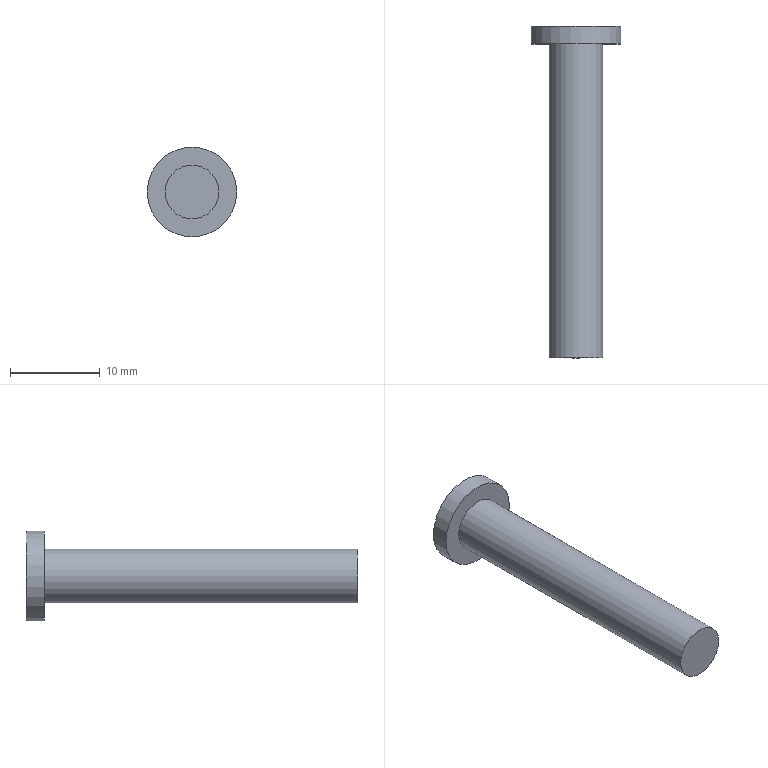Component | NX | SHE_JI-5 | 1 solid | 5 faces | box 10 x 37 x 10 mm | volume 1147 mm3 | plane 3 | cylinder 2 | commonest cylinder face diameters 6 x1 10 x1
STEP:
#1=CARTESIAN_POINT('',(0.,0.,0.));
#2=DIRECTION('',(0.,0.,1.));
#3=DIRECTION('',(1.,0.,0.));
#4=AXIS2_PLACEMENT_3D('',#1,#2,#3);
#5=CARTESIAN_POINT('',(-45.,-19.,20.));
#6=VERTEX_POINT('',#5);
#7=CARTESIAN_POINT('',(-48.,-19.,20.));
#8=DIRECTION('',(0.,1.,0.));
#9=DIRECTION('',(1.,0.,0.));
#10=AXIS2_PLACEMENT_3D('',#7,#8,#9);
#11=CIRCLE('',#10,3.);
#12=CARTESIAN_POINT('',(-48.,-19.,20.));
#13=DIRECTION('',(0.,-1.,0.));
#14=DIRECTION('',(1.,0.,0.));
#15=AXIS2_PLACEMENT_3D('',#12,#13,#14);
#16=PLANE('',#15);
#17=CARTESIAN_POINT('',(3.,0.));
#18=CARTESIAN_POINT('',(3.,-5.196));
#19=CARTESIAN_POINT('',(-1.5,-2.598));
#20=CARTESIAN_POINT('',(-6.,-0.));
#21=CARTESIAN_POINT('',(-1.5,2.598));
#22=CARTESIAN_POINT('',(3.,5.196));
#23=CARTESIAN_POINT('',(3.,0.));
#24=(BOUNDED_CURVE()B_SPLINE_CURVE(2,(#17,#18,#19,#20,#21,#22,#23),.UNSPECIFIED.,.T.,.F.)B_SPLINE_CURVE_WITH_KNOTS((1,2,2,2,2,1),(-2.094,0.,2.094,4.189,6.283,8.378),.UNSPECIFIED.)CURVE()GEOMETRIC_REPRESENTATION_ITEM()RATIONAL_B_SPLINE_CURVE((1.,0.5,1.,0.5,1.,0.5,1.))REPRESENTATION_ITEM(''));
#25=(GEOMETRIC_REPRESENTATION_CONTEXT(2)PARAMETRIC_REPRESENTATION_CONTEXT()REPRESENTATION_CONTEXT('',''));
#26=DEFINITIONAL_REPRESENTATION('',(#24),#25);
#27=PCURVE('',#16,#26);
#28=CARTESIAN_POINT('',(-48.,16.,20.));
#29=DIRECTION('',(0.,-1.,0.));
#30=DIRECTION('',(1.,0.,0.));
#31=AXIS2_PLACEMENT_3D('',#28,#29,#30);
#32=CYLINDRICAL_SURFACE('',#31,3.);
#33=CARTESIAN_POINT('',(6.283,35.));
#34=DIRECTION('',(-1.,0.));
#35=VECTOR('',#34,1.);
#36=LINE('',#33,#35);
#37=(GEOMETRIC_REPRESENTATION_CONTEXT(2)PARAMETRIC_REPRESENTATION_CONTEXT()REPRESENTATION_CONTEXT('',''));
#38=DEFINITIONAL_REPRESENTATION('',(#36),#37);
#39=PCURVE('',#32,#38);
#40=SURFACE_CURVE('',#11,(#27,#39),.PCURVE_S1.);
#41=EDGE_CURVE('',#6,#6,#40,.T.);
#42=ORIENTED_EDGE('',*,*,#41,.F.);
#43=EDGE_LOOP('',(#42));
#44=FACE_BOUND('',#43,.T.);
#45=ADVANCED_FACE('',(#44),#16,.T.);
#46=ORIENTED_EDGE('',*,*,#41,.T.);
#47=CARTESIAN_POINT('',(-45.,16.,20.));
#48=VERTEX_POINT('',#47);
#49=CARTESIAN_POINT('',(-45.,16.,20.));
#50=CARTESIAN_POINT('',(-45.,-19.,20.));
#51=B_SPLINE_CURVE_WITH_KNOTS('',1,(#49,#50),.UNSPECIFIED.,.F.,.F.,(2,2),(0.,35.),.PIECEWISE_BEZIER_KNOTS.);
#52=CARTESIAN_POINT('',(0.,0.));
#53=DIRECTION('',(0.,1.));
#54=VECTOR('',#53,1.);
#55=LINE('',#52,#54);
#56=(GEOMETRIC_REPRESENTATION_CONTEXT(2)PARAMETRIC_REPRESENTATION_CONTEXT()REPRESENTATION_CONTEXT('',''));
#57=DEFINITIONAL_REPRESENTATION('',(#55),#56);
#58=PCURVE('',#32,#57);
#59=CARTESIAN_POINT('',(6.283,0.));
#60=DIRECTION('',(0.,1.));
#61=VECTOR('',#60,1.);
#62=LINE('',#59,#61);
#63=(GEOMETRIC_REPRESENTATION_CONTEXT(2)PARAMETRIC_REPRESENTATION_CONTEXT()REPRESENTATION_CONTEXT('',''));
#64=DEFINITIONAL_REPRESENTATION('',(#62),#63);
#65=PCURVE('',#32,#64);
#66=SEAM_CURVE('',#51,(#58,#65),.PCURVE_S1.);
#67=EDGE_CURVE('',#48,#6,#66,.T.);
#68=ORIENTED_EDGE('',*,*,#67,.F.);
#69=CARTESIAN_POINT('',(-48.,16.,20.));
#70=DIRECTION('',(0.,-1.,0.));
#71=DIRECTION('',(1.,0.,0.));
#72=AXIS2_PLACEMENT_3D('',#69,#70,#71);
#73=CIRCLE('',#72,3.);
#74=CARTESIAN_POINT('',(0.,0.));
#75=DIRECTION('',(1.,0.));
#76=VECTOR('',#75,1.);
#77=LINE('',#74,#76);
#78=(GEOMETRIC_REPRESENTATION_CONTEXT(2)PARAMETRIC_REPRESENTATION_CONTEXT()REPRESENTATION_CONTEXT('',''));
#79=DEFINITIONAL_REPRESENTATION('',(#77),#78);
#80=PCURVE('',#32,#79);
#81=CARTESIAN_POINT('',(-48.,16.,20.));
#82=DIRECTION('',(0.,-1.,0.));
#83=DIRECTION('',(1.,0.,0.));
#84=AXIS2_PLACEMENT_3D('',#81,#82,#83);
#85=PLANE('',#84);
#86=CARTESIAN_POINT('',(0.,0.));
#87=DIRECTION('',(1.,0.));
#88=AXIS2_PLACEMENT_2D('',#86,#87);
#89=CIRCLE('',#88,3.);
#90=(GEOMETRIC_REPRESENTATION_CONTEXT(2)PARAMETRIC_REPRESENTATION_CONTEXT()REPRESENTATION_CONTEXT('',''));
#91=DEFINITIONAL_REPRESENTATION('',(#89),#90);
#92=PCURVE('',#85,#91);
#93=SURFACE_CURVE('',#73,(#80,#92),.PCURVE_S1.);
#94=EDGE_CURVE('',#48,#48,#93,.T.);
#95=ORIENTED_EDGE('',*,*,#94,.T.);
#96=ORIENTED_EDGE('',*,*,#67,.T.);
#97=EDGE_LOOP('',(#46,#68,#95,#96));
#98=FACE_BOUND('',#97,.T.);
#99=ADVANCED_FACE('',(#98),#32,.T.);
#100=CARTESIAN_POINT('',(-43.,18.,20.));
#101=VERTEX_POINT('',#100);
#102=CARTESIAN_POINT('',(-48.,18.,20.));
#103=DIRECTION('',(0.,-1.,0.));
#104=DIRECTION('',(1.,0.,0.));
#105=AXIS2_PLACEMENT_3D('',#102,#103,#104);
#106=CIRCLE('',#105,5.);
#107=CARTESIAN_POINT('',(-48.,18.,20.));
#108=DIRECTION('',(0.,1.,0.));
#109=DIRECTION('',(-1.,0.,0.));
#110=AXIS2_PLACEMENT_3D('',#107,#108,#109);
#111=PLANE('',#110);
#112=CARTESIAN_POINT('',(-5.,0.));
#113=CARTESIAN_POINT('',(-5.,8.66));
#114=CARTESIAN_POINT('',(2.5,4.33));
#115=CARTESIAN_POINT('',(10.,0.));
#116=CARTESIAN_POINT('',(2.5,-4.33));
#117=CARTESIAN_POINT('',(-5.,-8.66));
#118=CARTESIAN_POINT('',(-5.,0.));
#119=(BOUNDED_CURVE()B_SPLINE_CURVE(2,(#112,#113,#114,#115,#116,#117,#118),.UNSPECIFIED.,.T.,.F.)B_SPLINE_CURVE_WITH_KNOTS((1,2,2,2,2,1),(-2.094,0.,2.094,4.189,6.283,8.378),.UNSPECIFIED.)CURVE()GEOMETRIC_REPRESENTATION_ITEM()RATIONAL_B_SPLINE_CURVE((1.,0.5,1.,0.5,1.,0.5,1.))REPRESENTATION_ITEM(''));
#120=(GEOMETRIC_REPRESENTATION_CONTEXT(2)PARAMETRIC_REPRESENTATION_CONTEXT()REPRESENTATION_CONTEXT('',''));
#121=DEFINITIONAL_REPRESENTATION('',(#119),#120);
#122=PCURVE('',#111,#121);
#123=CARTESIAN_POINT('',(-48.,16.,20.));
#124=DIRECTION('',(0.,1.,0.));
#125=DIRECTION('',(1.,0.,0.));
#126=AXIS2_PLACEMENT_3D('',#123,#124,#125);
#127=CYLINDRICAL_SURFACE('',#126,5.);
#128=CARTESIAN_POINT('',(6.283,2.));
#129=DIRECTION('',(-1.,0.));
#130=VECTOR('',#129,1.);
#131=LINE('',#128,#130);
#132=(GEOMETRIC_REPRESENTATION_CONTEXT(2)PARAMETRIC_REPRESENTATION_CONTEXT()REPRESENTATION_CONTEXT('',''));
#133=DEFINITIONAL_REPRESENTATION('',(#131),#132);
#134=PCURVE('',#127,#133);
#135=SURFACE_CURVE('',#106,(#122,#134),.PCURVE_S1.);
#136=EDGE_CURVE('',#101,#101,#135,.T.);
#137=ORIENTED_EDGE('',*,*,#136,.F.);
#138=EDGE_LOOP('',(#137));
#139=FACE_BOUND('',#138,.T.);
#140=ADVANCED_FACE('',(#139),#111,.T.);
#141=ORIENTED_EDGE('',*,*,#94,.F.);
#142=EDGE_LOOP('',(#141));
#143=FACE_BOUND('',#142,.T.);
#144=CARTESIAN_POINT('',(-43.,16.,20.));
#145=VERTEX_POINT('',#144);
#146=CARTESIAN_POINT('',(-48.,16.,20.));
#147=DIRECTION('',(0.,1.,0.));
#148=DIRECTION('',(1.,0.,0.));
#149=AXIS2_PLACEMENT_3D('',#146,#147,#148);
#150=CIRCLE('',#149,5.);
#151=CARTESIAN_POINT('',(5.,0.));
#152=CARTESIAN_POINT('',(5.,-8.66));
#153=CARTESIAN_POINT('',(-2.5,-4.33));
#154=CARTESIAN_POINT('',(-10.,-0.));
#155=CARTESIAN_POINT('',(-2.5,4.33));
#156=CARTESIAN_POINT('',(5.,8.66));
#157=CARTESIAN_POINT('',(5.,0.));
#158=(BOUNDED_CURVE()B_SPLINE_CURVE(2,(#151,#152,#153,#154,#155,#156,#157),.UNSPECIFIED.,.T.,.F.)B_SPLINE_CURVE_WITH_KNOTS((1,2,2,2,2,1),(-2.094,0.,2.094,4.189,6.283,8.378),.UNSPECIFIED.)CURVE()GEOMETRIC_REPRESENTATION_ITEM()RATIONAL_B_SPLINE_CURVE((1.,0.5,1.,0.5,1.,0.5,1.))REPRESENTATION_ITEM(''));
#159=(GEOMETRIC_REPRESENTATION_CONTEXT(2)PARAMETRIC_REPRESENTATION_CONTEXT()REPRESENTATION_CONTEXT('',''));
#160=DEFINITIONAL_REPRESENTATION('',(#158),#159);
#161=PCURVE('',#85,#160);
#162=CARTESIAN_POINT('',(0.,0.));
#163=DIRECTION('',(1.,0.));
#164=VECTOR('',#163,1.);
#165=LINE('',#162,#164);
#166=(GEOMETRIC_REPRESENTATION_CONTEXT(2)PARAMETRIC_REPRESENTATION_CONTEXT()REPRESENTATION_CONTEXT('',''));
#167=DEFINITIONAL_REPRESENTATION('',(#165),#166);
#168=PCURVE('',#127,#167);
#169=SURFACE_CURVE('',#150,(#161,#168),.PCURVE_S1.);
#170=EDGE_CURVE('',#145,#145,#169,.T.);
#171=ORIENTED_EDGE('',*,*,#170,.F.);
#172=EDGE_LOOP('',(#171));
#173=FACE_BOUND('',#172,.T.);
#174=ADVANCED_FACE('',(#143,#173),#85,.T.);
#175=ORIENTED_EDGE('',*,*,#136,.T.);
#176=CARTESIAN_POINT('',(-43.,16.,20.));
#177=CARTESIAN_POINT('',(-43.,18.,20.));
#178=B_SPLINE_CURVE_WITH_KNOTS('',1,(#176,#177),.UNSPECIFIED.,.F.,.F.,(2,2),(0.,2.),.PIECEWISE_BEZIER_KNOTS.);
#179=CARTESIAN_POINT('',(0.,0.));
#180=DIRECTION('',(0.,1.));
#181=VECTOR('',#180,1.);
#182=LINE('',#179,#181);
#183=(GEOMETRIC_REPRESENTATION_CONTEXT(2)PARAMETRIC_REPRESENTATION_CONTEXT()REPRESENTATION_CONTEXT('',''));
#184=DEFINITIONAL_REPRESENTATION('',(#182),#183);
#185=PCURVE('',#127,#184);
#186=CARTESIAN_POINT('',(6.283,0.));
#187=DIRECTION('',(0.,1.));
#188=VECTOR('',#187,1.);
#189=LINE('',#186,#188);
#190=(GEOMETRIC_REPRESENTATION_CONTEXT(2)PARAMETRIC_REPRESENTATION_CONTEXT()REPRESENTATION_CONTEXT('',''));
#191=DEFINITIONAL_REPRESENTATION('',(#189),#190);
#192=PCURVE('',#127,#191);
#193=SEAM_CURVE('',#178,(#185,#192),.PCURVE_S1.);
#194=EDGE_CURVE('',#145,#101,#193,.T.);
#195=ORIENTED_EDGE('',*,*,#194,.F.);
#196=ORIENTED_EDGE('',*,*,#170,.T.);
#197=ORIENTED_EDGE('',*,*,#194,.T.);
#198=EDGE_LOOP('',(#175,#195,#196,#197));
#199=FACE_BOUND('',#198,.T.);
#200=ADVANCED_FACE('',(#199),#127,.T.);
#201=CLOSED_SHELL('',(#45,#99,#140,#174,#200));
#202=MANIFOLD_SOLID_BREP('',#201);
#203=(LENGTH_UNIT()NAMED_UNIT(*)SI_UNIT(.MILLI.,.METRE.));
#204=UNCERTAINTY_MEASURE_WITH_UNIT(LENGTH_MEASURE(0.00001),#203,'','');
#205=(NAMED_UNIT(*)PLANE_ANGLE_UNIT()SI_UNIT($,.RADIAN.));
#206=(NAMED_UNIT(*)SI_UNIT($,.STERADIAN.)SOLID_ANGLE_UNIT());
#207=(GEOMETRIC_REPRESENTATION_CONTEXT(3)GLOBAL_UNCERTAINTY_ASSIGNED_CONTEXT((#204))GLOBAL_UNIT_ASSIGNED_CONTEXT((#203,#205,#206))REPRESENTATION_CONTEXT('',''));
#208=ADVANCED_BREP_SHAPE_REPRESENTATION('',(#4,#202),#207);